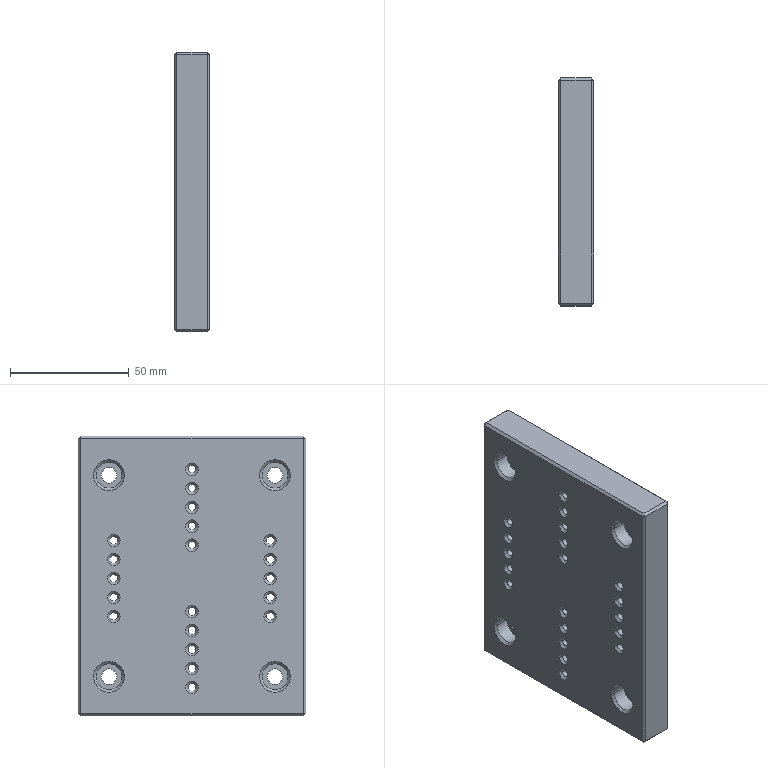Component | SolidWorks | ShimPlate4-1 | 1 solid | 182 faces | box 15 x 96 x 118 mm | volume 162826 mm3 | cone 96 | cylinder 56 | plane 30 | commonest cylinder face diameters 3.3 x40 11 x8 6.6 x8 | material 1060 Alloy
build123d program:
from build123d import *

# Parameters (mm, degrees)
SKETCH1_W                                          = 96
SKETCH1_H                                          = 118
BOSS_EXTRUDE1_DEPTH                                = 15
HOLE_SIZE_ACCORDING_TO_TYPE_OF_HEXAGON_D           = 6.6
HOLE_SIZE_ACCORDING_TO_TYPE_OF_HEXAGON_CBORE_D     = 11
HOLE_SIZE_ACCORDING_TO_TYPE_OF_HEXAGON_CBORE_DEPTH = 6.8
M4_TAPPED_HOLE1_D                                  = 3.3
LPATTERN2_COUNT                                    = 3
LPATTERN2_PITCH                                    = 8
LPATTERN3_COUNT                                    = 3
LPATTERN3_PITCH                                    = 8
CHAMFER1_SIZE                                      = 1


with BuildPart() as part:
    # Sketch1 → Boss-Extrude1 (new body)
    with BuildSketch(Plane.XY):
        Rectangle(SKETCH1_W, SKETCH1_H)
    extrude(amount=BOSS_EXTRUDE1_DEPTH)

    # Hole Size _according to_ type of Hexagon (through all)
    with Locations(Plane.XY.offset(15)):
        with Locations((-35, 42.5), (35, 42.5), (35, -42.5), (-35, -42.5)):
            CounterBoreHole(HOLE_SIZE_ACCORDING_TO_TYPE_OF_HEXAGON_D / 2, HOLE_SIZE_ACCORDING_TO_TYPE_OF_HEXAGON_CBORE_D / 2, HOLE_SIZE_ACCORDING_TO_TYPE_OF_HEXAGON_CBORE_DEPTH)

    # M4 Tapped Hole1 (through all)
    with Locations(Plane.XY.offset(15)):
        with Locations((0, 29), (0, -31), (33, -1), (-33, -1)):
            m4_tapped_hole1 = Hole(M4_TAPPED_HOLE1_D / 2)

    # LPattern2: M4 Tapped Hole1 ×3
    with Locations(*[(0, -i * LPATTERN2_PITCH, 0) for i in range(1, LPATTERN2_COUNT)]):
        add(m4_tapped_hole1, mode=Mode.SUBTRACT)

    # LPattern3: M4 Tapped Hole1 ×3
    with Locations(*[(0, i * LPATTERN3_PITCH, 0) for i in range(1, LPATTERN3_COUNT)]):
        add(m4_tapped_hole1, mode=Mode.SUBTRACT)

    # Chamfer1
    chamfer1_edges = [part.edges().sort_by_distance(p)[0] for p in [
        (48, 0, 15),
        (-31.35, 7, 15),
        (-31.35, 7, 0),
        (-31.35, 15, 0),
        (-31.35, 15, 15),
        (34.65, 7, 15),
        (34.65, 7, 0),
        (34.65, 15, 0),
        (34.65, 15, 15),
        (1.65, -23, 15),
        (1.65, -23, 0),
        (1.65, -15, 0),
        (1.65, -15, 15),
        (0, 59, 15),
        (-40.5, -42.5, 15),
        (-31.7, -42.5, 0),
        (29.5, -42.5, 15),
        (38.3, -42.5, 0),
        (29.5, 42.5, 15),
        (38.3, 42.5, 0),
        (-40.5, 42.5, 15),
        (-31.7, 42.5, 0),
        (-48, 0, 15),
        (0, 59, 0),
        (-31.35, -1, 15),
        (-31.35, -1, 0),
        (48, 0, 0),
        (34.65, -1, 15),
        (34.65, -1, 0),
        (0, -59, 0),
        (-48, 0, 0),
        (1.65, -31, 15),
        (1.65, -31, 0),
        (1.65, 29, 15),
        (1.65, 29, 0),
        (1.65, 21, 15),
        (1.65, 21, 0),
        (0, -59, 15),
        (1.65, 13, 0),
        (1.65, 13, 15),
        (-48, 59, 7.5),
        (48, 59, 7.5),
        (-31.35, -9, 15),
        (-31.35, -9, 0),
        (48, -59, 7.5),
        (-48, -59, 7.5),
        (-31.35, -17, 0),
        (-31.35, -17, 15),
        (34.65, -9, 15),
        (34.65, -9, 0),
        (34.65, -17, 0),
        (34.65, -17, 15),
        (1.65, -39, 15),
        (1.65, -39, 0),
        (1.65, -47, 0),
        (1.65, -47, 15),
        (1.65, 37, 15),
        (1.65, 37, 0),
        (1.65, 45, 0),
        (1.65, 45, 15),
    ]]
    chamfer(chamfer1_edges, length=CHAMFER1_SIZE)


solid = part.part

# Placed as in the assembly
solid = solid.moved(Location((-164.666, 347.264, -100), (90, -90, 0)))